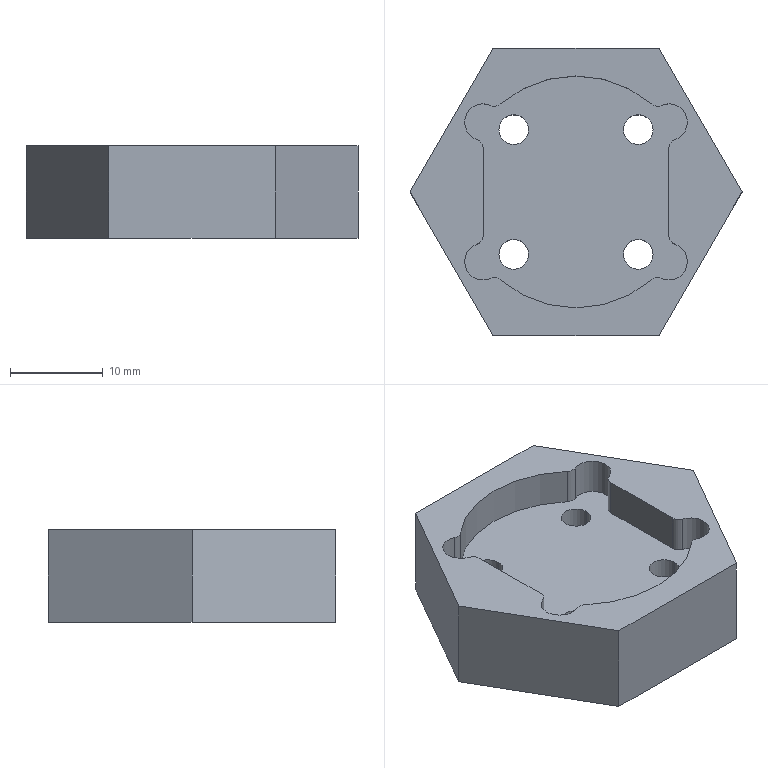CAM job | Mastercam | mm | 11 operations | part box 420 x 297 x 10
1. Facing | 20 - 63 平铣刀
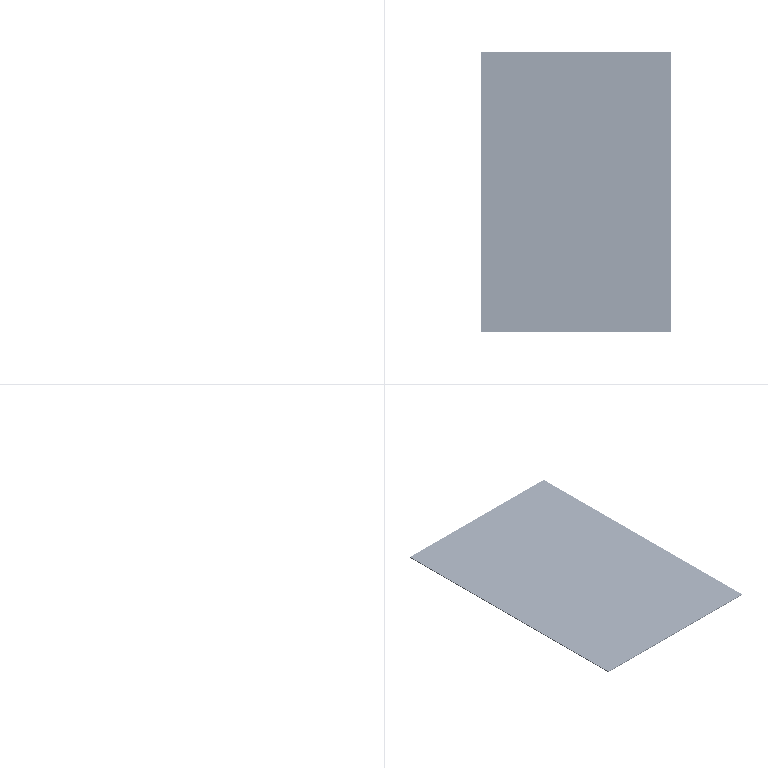2. 2D High Speed (2D Dynamic Mill) | 10 - 10 平铣刀
3. Contour (2D) | 10 - 10 平铣刀
4. 2D High Speed (2D Area Mill) | 3 - 3 平铣刀
5. Contour (2D) | 3 - 3 平铣刀
6. Drill/Counterbore | 7 - 4 倒角刀
7. Contour (2D chamfer) | 7 - 4 倒角刀
8. Facing | 20 - 63 平铣刀
9. Contour (2D chamfer) | 7 - 4 倒角刀
10. Drill/Counterbore | 7 - 4 倒角刀
11. Peck Drill | 1 - 4.2 钻头